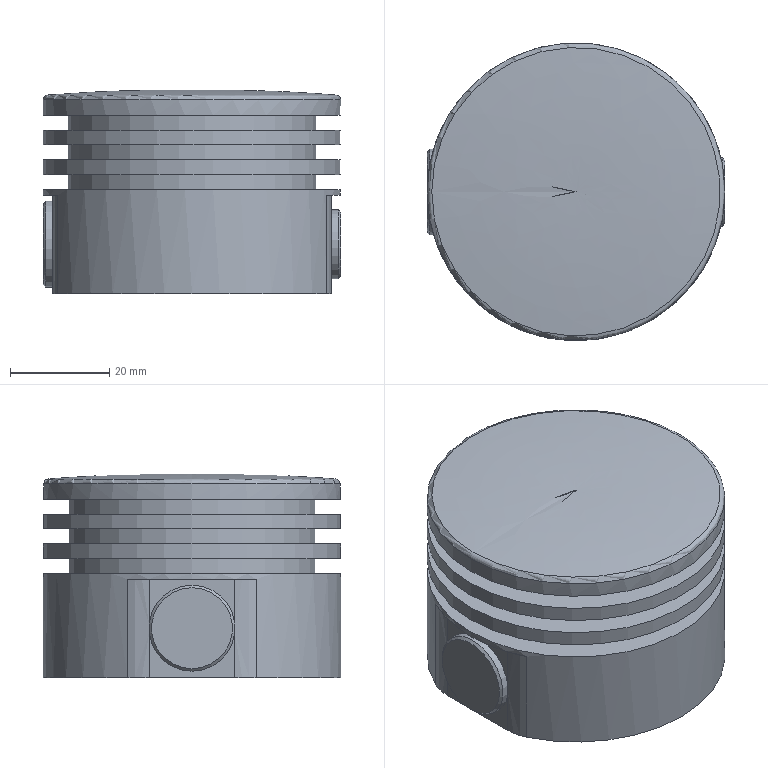Component | NX | PISTON_3 | 2 solids | 37 faces | volume 60051 mm3 | cylinder 17 | plane 15 | cone 3 | spline 1 | torus 1 | commonest cylinder face diameters 60 x4 20 x4 50 x3 13.95 x3 46 x1 40 x1 17.344 x1